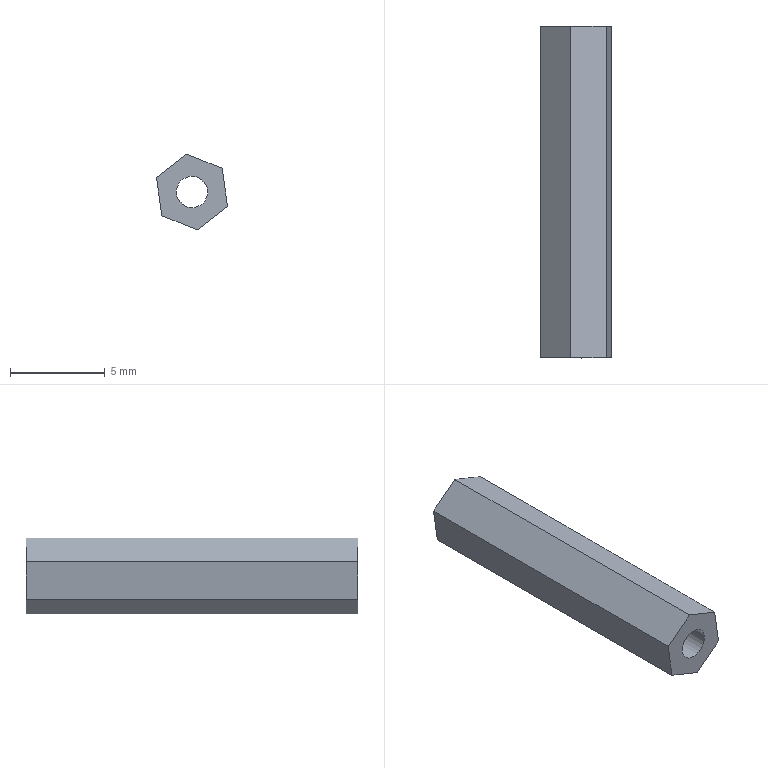Component | NX | 13 | 1 solid | 9 faces | box 3.75 x 17.5 x 4 mm | volume 148 mm3 | plane 8 | cylinder 1 | commonest cylinder face diameters 1.65 x1
STEP:
#1=CARTESIAN_POINT('',(0.,0.,0.));
#2=DIRECTION('',(0.,0.,1.));
#3=DIRECTION('',(1.,0.,0.));
#4=AXIS2_PLACEMENT_3D('',#1,#2,#3);
#5=CARTESIAN_POINT('',(-512.048,186.249,-204.937));
#6=VERTEX_POINT('',#5);
#7=CARTESIAN_POINT('',(-512.048,168.749,-204.937));
#8=VERTEX_POINT('',#7);
#9=CARTESIAN_POINT('',(-512.048,168.749,-204.937));
#10=DIRECTION('',(0.,-1.,0.));
#11=VECTOR('',#10,1.);
#12=LINE('',#9,#11);
#13=CARTESIAN_POINT('',(-510.174,168.749,-205.694));
#14=DIRECTION('',(-0.3746,0.,-0.9272));
#15=DIRECTION('',(-0.9272,0.,0.3746));
#16=AXIS2_PLACEMENT_3D('',#13,#14,#15);
#17=PLANE('',#16);
#18=CARTESIAN_POINT('',(2.021,0.));
#19=DIRECTION('',(0.,-1.));
#20=VECTOR('',#19,1.);
#21=LINE('',#18,#20);
#22=(GEOMETRIC_REPRESENTATION_CONTEXT(2)PARAMETRIC_REPRESENTATION_CONTEXT()REPRESENTATION_CONTEXT('',''));
#23=DEFINITIONAL_REPRESENTATION('',(#21),#22);
#24=PCURVE('',#17,#23);
#25=CARTESIAN_POINT('',(-512.048,168.749,-204.937));
#26=DIRECTION('',(0.6157,0.,-0.788));
#27=DIRECTION('',(0.,-1.,0.));
#28=AXIS2_PLACEMENT_3D('',#25,#26,#27);
#29=PLANE('',#28);
#30=CARTESIAN_POINT('',(0.,0.));
#31=DIRECTION('',(1.,0.));
#32=VECTOR('',#31,1.);
#33=LINE('',#30,#32);
#34=(GEOMETRIC_REPRESENTATION_CONTEXT(2)PARAMETRIC_REPRESENTATION_CONTEXT()REPRESENTATION_CONTEXT('',''));
#35=DEFINITIONAL_REPRESENTATION('',(#33),#34);
#36=PCURVE('',#29,#35);
#37=SURFACE_CURVE('',#12,(#24,#36),.PCURVE_S1.);
#38=EDGE_CURVE('',#6,#8,#37,.T.);
#39=ORIENTED_EDGE('',*,*,#38,.T.);
#40=CARTESIAN_POINT('',(-510.174,168.749,-205.694));
#41=VERTEX_POINT('',#40);
#42=CARTESIAN_POINT('',(-510.174,168.749,-205.694));
#43=DIRECTION('',(-0.9272,0.,0.3746));
#44=VECTOR('',#43,1.);
#45=LINE('',#42,#44);
#46=CARTESIAN_POINT('',(0.,0.));
#47=DIRECTION('',(1.,0.));
#48=VECTOR('',#47,1.);
#49=LINE('',#46,#48);
#50=(GEOMETRIC_REPRESENTATION_CONTEXT(2)PARAMETRIC_REPRESENTATION_CONTEXT()REPRESENTATION_CONTEXT('',''));
#51=DEFINITIONAL_REPRESENTATION('',(#49),#50);
#52=PCURVE('',#17,#51);
#53=CARTESIAN_POINT('',(-511.767,168.749,-206.939));
#54=DIRECTION('',(0.,-1.,0.));
#55=DIRECTION('',(-0.788,0.,-0.6157));
#56=AXIS2_PLACEMENT_3D('',#53,#54,#55);
#57=PLANE('',#56);
#58=CARTESIAN_POINT('',(-2.021,0.));
#59=DIRECTION('',(0.5,-0.866));
#60=VECTOR('',#59,1.);
#61=LINE('',#58,#60);
#62=(GEOMETRIC_REPRESENTATION_CONTEXT(2)PARAMETRIC_REPRESENTATION_CONTEXT()REPRESENTATION_CONTEXT('',''));
#63=DEFINITIONAL_REPRESENTATION('',(#61),#62);
#64=PCURVE('',#57,#63);
#65=SURFACE_CURVE('',#45,(#52,#64),.PCURVE_S1.);
#66=EDGE_CURVE('',#41,#8,#65,.T.);
#67=ORIENTED_EDGE('',*,*,#66,.F.);
#68=CARTESIAN_POINT('',(-510.174,186.249,-205.694));
#69=VERTEX_POINT('',#68);
#70=CARTESIAN_POINT('',(-510.174,168.749,-205.694));
#71=DIRECTION('',(0.,1.,0.));
#72=VECTOR('',#71,1.);
#73=LINE('',#70,#72);
#74=CARTESIAN_POINT('',(0.,0.));
#75=DIRECTION('',(0.,1.));
#76=VECTOR('',#75,1.);
#77=LINE('',#74,#76);
#78=(GEOMETRIC_REPRESENTATION_CONTEXT(2)PARAMETRIC_REPRESENTATION_CONTEXT()REPRESENTATION_CONTEXT('',''));
#79=DEFINITIONAL_REPRESENTATION('',(#77),#78);
#80=PCURVE('',#17,#79);
#81=CARTESIAN_POINT('',(-509.893,168.749,-207.695));
#82=DIRECTION('',(-0.9903,0.,-0.1392));
#83=DIRECTION('',(-0.1392,0.,0.9903));
#84=AXIS2_PLACEMENT_3D('',#81,#82,#83);
#85=PLANE('',#84);
#86=CARTESIAN_POINT('',(2.021,0.));
#87=DIRECTION('',(0.,1.));
#88=VECTOR('',#87,1.);
#89=LINE('',#86,#88);
#90=(GEOMETRIC_REPRESENTATION_CONTEXT(2)PARAMETRIC_REPRESENTATION_CONTEXT()REPRESENTATION_CONTEXT('',''));
#91=DEFINITIONAL_REPRESENTATION('',(#89),#90);
#92=PCURVE('',#85,#91);
#93=SURFACE_CURVE('',#73,(#80,#92),.PCURVE_S1.);
#94=EDGE_CURVE('',#41,#69,#93,.T.);
#95=ORIENTED_EDGE('',*,*,#94,.T.);
#96=CARTESIAN_POINT('',(-510.174,186.249,-205.694));
#97=DIRECTION('',(-0.9272,0.,0.3746));
#98=VECTOR('',#97,1.);
#99=LINE('',#96,#98);
#100=CARTESIAN_POINT('',(0.,17.5));
#101=DIRECTION('',(1.,0.));
#102=VECTOR('',#101,1.);
#103=LINE('',#100,#102);
#104=(GEOMETRIC_REPRESENTATION_CONTEXT(2)PARAMETRIC_REPRESENTATION_CONTEXT()REPRESENTATION_CONTEXT('',''));
#105=DEFINITIONAL_REPRESENTATION('',(#103),#104);
#106=PCURVE('',#17,#105);
#107=CARTESIAN_POINT('',(-511.767,186.249,-206.939));
#108=DIRECTION('',(0.,-1.,0.));
#109=DIRECTION('',(-0.788,0.,-0.6157));
#110=AXIS2_PLACEMENT_3D('',#107,#108,#109);
#111=PLANE('',#110);
#112=CARTESIAN_POINT('',(-2.021,0.));
#113=DIRECTION('',(0.5,-0.866));
#114=VECTOR('',#113,1.);
#115=LINE('',#112,#114);
#116=(GEOMETRIC_REPRESENTATION_CONTEXT(2)PARAMETRIC_REPRESENTATION_CONTEXT()REPRESENTATION_CONTEXT('',''));
#117=DEFINITIONAL_REPRESENTATION('',(#115),#116);
#118=PCURVE('',#111,#117);
#119=SURFACE_CURVE('',#99,(#106,#118),.PCURVE_S1.);
#120=EDGE_CURVE('',#69,#6,#119,.T.);
#121=ORIENTED_EDGE('',*,*,#120,.T.);
#122=EDGE_LOOP('',(#39,#67,#95,#121));
#123=FACE_BOUND('',#122,.T.);
#124=ADVANCED_FACE('',(#123),#17,.F.);
#125=CARTESIAN_POINT('',(-513.64,186.249,-206.182));
#126=VERTEX_POINT('',#125);
#127=CARTESIAN_POINT('',(-513.64,168.749,-206.182));
#128=VERTEX_POINT('',#127);
#129=CARTESIAN_POINT('',(-513.64,168.749,-206.182));
#130=DIRECTION('',(0.,-1.,0.));
#131=VECTOR('',#130,1.);
#132=LINE('',#129,#131);
#133=CARTESIAN_POINT('',(0.,2.021));
#134=DIRECTION('',(1.,0.));
#135=VECTOR('',#134,1.);
#136=LINE('',#133,#135);
#137=(GEOMETRIC_REPRESENTATION_CONTEXT(2)PARAMETRIC_REPRESENTATION_CONTEXT()REPRESENTATION_CONTEXT('',''));
#138=DEFINITIONAL_REPRESENTATION('',(#136),#137);
#139=PCURVE('',#29,#138);
#140=CARTESIAN_POINT('',(-513.64,168.749,-206.182));
#141=DIRECTION('',(0.9903,0.,0.1392));
#142=DIRECTION('',(0.1392,0.,-0.9903));
#143=AXIS2_PLACEMENT_3D('',#140,#141,#142);
#144=PLANE('',#143);
#145=CARTESIAN_POINT('',(0.,0.));
#146=DIRECTION('',(0.,-1.));
#147=VECTOR('',#146,1.);
#148=LINE('',#145,#147);
#149=(GEOMETRIC_REPRESENTATION_CONTEXT(2)PARAMETRIC_REPRESENTATION_CONTEXT()REPRESENTATION_CONTEXT('',''));
#150=DEFINITIONAL_REPRESENTATION('',(#148),#149);
#151=PCURVE('',#144,#150);
#152=SURFACE_CURVE('',#132,(#139,#151),.PCURVE_S1.);
#153=EDGE_CURVE('',#126,#128,#152,.T.);
#154=ORIENTED_EDGE('',*,*,#153,.T.);
#155=CARTESIAN_POINT('',(-512.844,168.749,-205.559));
#156=DIRECTION('',(-0.788,0.,-0.6157));
#157=VECTOR('',#156,1.);
#158=LINE('',#155,#157);
#159=CARTESIAN_POINT('',(0.,1.01));
#160=DIRECTION('',(0.,1.));
#161=VECTOR('',#160,1.);
#162=LINE('',#159,#161);
#163=(GEOMETRIC_REPRESENTATION_CONTEXT(2)PARAMETRIC_REPRESENTATION_CONTEXT()REPRESENTATION_CONTEXT('',''));
#164=DEFINITIONAL_REPRESENTATION('',(#162),#163);
#165=PCURVE('',#29,#164);
#166=CARTESIAN_POINT('',(0.,-1.75));
#167=DIRECTION('',(1.,0.));
#168=VECTOR('',#167,1.);
#169=LINE('',#166,#168);
#170=(GEOMETRIC_REPRESENTATION_CONTEXT(2)PARAMETRIC_REPRESENTATION_CONTEXT()REPRESENTATION_CONTEXT('',''));
#171=DEFINITIONAL_REPRESENTATION('',(#169),#170);
#172=PCURVE('',#57,#171);
#173=SURFACE_CURVE('',#158,(#165,#172),.PCURVE_S1.);
#174=EDGE_CURVE('',#8,#128,#173,.T.);
#175=ORIENTED_EDGE('',*,*,#174,.F.);
#176=ORIENTED_EDGE('',*,*,#38,.F.);
#177=CARTESIAN_POINT('',(-512.844,186.249,-205.559));
#178=DIRECTION('',(-0.788,0.,-0.6157));
#179=VECTOR('',#178,1.);
#180=LINE('',#177,#179);
#181=CARTESIAN_POINT('',(-17.5,1.01));
#182=DIRECTION('',(0.,1.));
#183=VECTOR('',#182,1.);
#184=LINE('',#181,#183);
#185=(GEOMETRIC_REPRESENTATION_CONTEXT(2)PARAMETRIC_REPRESENTATION_CONTEXT()REPRESENTATION_CONTEXT('',''));
#186=DEFINITIONAL_REPRESENTATION('',(#184),#185);
#187=PCURVE('',#29,#186);
#188=CARTESIAN_POINT('',(0.,-1.75));
#189=DIRECTION('',(1.,0.));
#190=VECTOR('',#189,1.);
#191=LINE('',#188,#190);
#192=(GEOMETRIC_REPRESENTATION_CONTEXT(2)PARAMETRIC_REPRESENTATION_CONTEXT()REPRESENTATION_CONTEXT('',''));
#193=DEFINITIONAL_REPRESENTATION('',(#191),#192);
#194=PCURVE('',#111,#193);
#195=SURFACE_CURVE('',#180,(#187,#194),.PCURVE_S1.);
#196=EDGE_CURVE('',#6,#126,#195,.T.);
#197=ORIENTED_EDGE('',*,*,#196,.T.);
#198=EDGE_LOOP('',(#154,#175,#176,#197));
#199=FACE_BOUND('',#198,.T.);
#200=ADVANCED_FACE('',(#199),#29,.F.);
#201=CARTESIAN_POINT('',(-513.359,186.249,-208.183));
#202=VERTEX_POINT('',#201);
#203=CARTESIAN_POINT('',(-513.359,168.749,-208.183));
#204=VERTEX_POINT('',#203);
#205=CARTESIAN_POINT('',(-513.359,168.749,-208.183));
#206=DIRECTION('',(0.,-1.,0.));
#207=VECTOR('',#206,1.);
#208=LINE('',#205,#207);
#209=CARTESIAN_POINT('',(2.021,0.));
#210=DIRECTION('',(0.,-1.));
#211=VECTOR('',#210,1.);
#212=LINE('',#209,#211);
#213=(GEOMETRIC_REPRESENTATION_CONTEXT(2)PARAMETRIC_REPRESENTATION_CONTEXT()REPRESENTATION_CONTEXT('',''));
#214=DEFINITIONAL_REPRESENTATION('',(#212),#213);
#215=PCURVE('',#144,#214);
#216=CARTESIAN_POINT('',(-513.359,168.749,-208.183));
#217=DIRECTION('',(0.3746,0.,0.9272));
#218=DIRECTION('',(0.9272,0.,-0.3746));
#219=AXIS2_PLACEMENT_3D('',#216,#217,#218);
#220=PLANE('',#219);
#221=CARTESIAN_POINT('',(0.,0.));
#222=DIRECTION('',(0.,-1.));
#223=VECTOR('',#222,1.);
#224=LINE('',#221,#223);
#225=(GEOMETRIC_REPRESENTATION_CONTEXT(2)PARAMETRIC_REPRESENTATION_CONTEXT()REPRESENTATION_CONTEXT('',''));
#226=DEFINITIONAL_REPRESENTATION('',(#224),#225);
#227=PCURVE('',#220,#226);
#228=SURFACE_CURVE('',#208,(#215,#227),.PCURVE_S1.);
#229=EDGE_CURVE('',#202,#204,#228,.T.);
#230=ORIENTED_EDGE('',*,*,#229,.T.);
#231=CARTESIAN_POINT('',(-513.64,168.749,-206.182));
#232=DIRECTION('',(0.1392,0.,-0.9903));
#233=VECTOR('',#232,1.);
#234=LINE('',#231,#233);
#235=CARTESIAN_POINT('',(0.,0.));
#236=DIRECTION('',(1.,0.));
#237=VECTOR('',#236,1.);
#238=LINE('',#235,#237);
#239=(GEOMETRIC_REPRESENTATION_CONTEXT(2)PARAMETRIC_REPRESENTATION_CONTEXT()REPRESENTATION_CONTEXT('',''));
#240=DEFINITIONAL_REPRESENTATION('',(#238),#239);
#241=PCURVE('',#144,#240);
#242=CARTESIAN_POINT('',(1.01,-1.75));
#243=DIRECTION('',(0.5,0.866));
#244=VECTOR('',#243,1.);
#245=LINE('',#242,#244);
#246=(GEOMETRIC_REPRESENTATION_CONTEXT(2)PARAMETRIC_REPRESENTATION_CONTEXT()REPRESENTATION_CONTEXT('',''));
#247=DEFINITIONAL_REPRESENTATION('',(#245),#246);
#248=PCURVE('',#57,#247);
#249=SURFACE_CURVE('',#234,(#241,#248),.PCURVE_S1.);
#250=EDGE_CURVE('',#128,#204,#249,.T.);
#251=ORIENTED_EDGE('',*,*,#250,.F.);
#252=ORIENTED_EDGE('',*,*,#153,.F.);
#253=CARTESIAN_POINT('',(-513.64,186.249,-206.182));
#254=DIRECTION('',(0.1392,0.,-0.9903));
#255=VECTOR('',#254,1.);
#256=LINE('',#253,#255);
#257=CARTESIAN_POINT('',(0.,17.5));
#258=DIRECTION('',(1.,0.));
#259=VECTOR('',#258,1.);
#260=LINE('',#257,#259);
#261=(GEOMETRIC_REPRESENTATION_CONTEXT(2)PARAMETRIC_REPRESENTATION_CONTEXT()REPRESENTATION_CONTEXT('',''));
#262=DEFINITIONAL_REPRESENTATION('',(#260),#261);
#263=PCURVE('',#144,#262);
#264=CARTESIAN_POINT('',(1.01,-1.75));
#265=DIRECTION('',(0.5,0.866));
#266=VECTOR('',#265,1.);
#267=LINE('',#264,#266);
#268=(GEOMETRIC_REPRESENTATION_CONTEXT(2)PARAMETRIC_REPRESENTATION_CONTEXT()REPRESENTATION_CONTEXT('',''));
#269=DEFINITIONAL_REPRESENTATION('',(#267),#268);
#270=PCURVE('',#111,#269);
#271=SURFACE_CURVE('',#256,(#263,#270),.PCURVE_S1.);
#272=EDGE_CURVE('',#126,#202,#271,.T.);
#273=ORIENTED_EDGE('',*,*,#272,.T.);
#274=EDGE_LOOP('',(#230,#251,#252,#273));
#275=FACE_BOUND('',#274,.T.);
#276=ADVANCED_FACE('',(#275),#144,.F.);
#277=CARTESIAN_POINT('',(-511.485,186.249,-208.94));
#278=VERTEX_POINT('',#277);
#279=CARTESIAN_POINT('',(-511.485,168.749,-208.94));
#280=VERTEX_POINT('',#279);
#281=CARTESIAN_POINT('',(-511.485,168.749,-208.94));
#282=DIRECTION('',(0.,-1.,0.));
#283=VECTOR('',#282,1.);
#284=LINE('',#281,#283);
#285=CARTESIAN_POINT('',(2.021,0.));
#286=DIRECTION('',(0.,-1.));
#287=VECTOR('',#286,1.);
#288=LINE('',#285,#287);
#289=(GEOMETRIC_REPRESENTATION_CONTEXT(2)PARAMETRIC_REPRESENTATION_CONTEXT()REPRESENTATION_CONTEXT('',''));
#290=DEFINITIONAL_REPRESENTATION('',(#288),#289);
#291=PCURVE('',#220,#290);
#292=CARTESIAN_POINT('',(-511.485,168.749,-208.94));
#293=DIRECTION('',(-0.6157,0.,0.788));
#294=DIRECTION('',(0.788,0.,0.6157));
#295=AXIS2_PLACEMENT_3D('',#292,#293,#294);
#296=PLANE('',#295);
#297=CARTESIAN_POINT('',(0.,0.));
#298=DIRECTION('',(0.,-1.));
#299=VECTOR('',#298,1.);
#300=LINE('',#297,#299);
#301=(GEOMETRIC_REPRESENTATION_CONTEXT(2)PARAMETRIC_REPRESENTATION_CONTEXT()REPRESENTATION_CONTEXT('',''));
#302=DEFINITIONAL_REPRESENTATION('',(#300),#301);
#303=PCURVE('',#296,#302);
#304=SURFACE_CURVE('',#284,(#291,#303),.PCURVE_S1.);
#305=EDGE_CURVE('',#278,#280,#304,.T.);
#306=ORIENTED_EDGE('',*,*,#305,.T.);
#307=CARTESIAN_POINT('',(-513.359,168.749,-208.183));
#308=DIRECTION('',(0.9272,0.,-0.3746));
#309=VECTOR('',#308,1.);
#310=LINE('',#307,#309);
#311=CARTESIAN_POINT('',(0.,0.));
#312=DIRECTION('',(1.,0.));
#313=VECTOR('',#312,1.);
#314=LINE('',#311,#313);
#315=(GEOMETRIC_REPRESENTATION_CONTEXT(2)PARAMETRIC_REPRESENTATION_CONTEXT()REPRESENTATION_CONTEXT('',''));
#316=DEFINITIONAL_REPRESENTATION('',(#314),#315);
#317=PCURVE('',#220,#316);
#318=CARTESIAN_POINT('',(2.021,0.));
#319=DIRECTION('',(-0.5,0.866));
#320=VECTOR('',#319,1.);
#321=LINE('',#318,#320);
#322=(GEOMETRIC_REPRESENTATION_CONTEXT(2)PARAMETRIC_REPRESENTATION_CONTEXT()REPRESENTATION_CONTEXT('',''));
#323=DEFINITIONAL_REPRESENTATION('',(#321),#322);
#324=PCURVE('',#57,#323);
#325=SURFACE_CURVE('',#310,(#317,#324),.PCURVE_S1.);
#326=EDGE_CURVE('',#204,#280,#325,.T.);
#327=ORIENTED_EDGE('',*,*,#326,.F.);
#328=ORIENTED_EDGE('',*,*,#229,.F.);
#329=CARTESIAN_POINT('',(-513.359,186.249,-208.183));
#330=DIRECTION('',(0.9272,0.,-0.3746));
#331=VECTOR('',#330,1.);
#332=LINE('',#329,#331);
#333=CARTESIAN_POINT('',(0.,17.5));
#334=DIRECTION('',(1.,0.));
#335=VECTOR('',#334,1.);
#336=LINE('',#333,#335);
#337=(GEOMETRIC_REPRESENTATION_CONTEXT(2)PARAMETRIC_REPRESENTATION_CONTEXT()REPRESENTATION_CONTEXT('',''));
#338=DEFINITIONAL_REPRESENTATION('',(#336),#337);
#339=PCURVE('',#220,#338);
#340=CARTESIAN_POINT('',(2.021,0.));
#341=DIRECTION('',(-0.5,0.866));
#342=VECTOR('',#341,1.);
#343=LINE('',#340,#342);
#344=(GEOMETRIC_REPRESENTATION_CONTEXT(2)PARAMETRIC_REPRESENTATION_CONTEXT()REPRESENTATION_CONTEXT('',''));
#345=DEFINITIONAL_REPRESENTATION('',(#343),#344);
#346=PCURVE('',#111,#345);
#347=SURFACE_CURVE('',#332,(#339,#346),.PCURVE_S1.);
#348=EDGE_CURVE('',#202,#278,#347,.T.);
#349=ORIENTED_EDGE('',*,*,#348,.T.);
#350=EDGE_LOOP('',(#306,#327,#328,#349));
#351=FACE_BOUND('',#350,.T.);
#352=ADVANCED_FACE('',(#351),#220,.F.);
#353=CARTESIAN_POINT('',(-509.893,186.249,-207.695));
#354=VERTEX_POINT('',#353);
#355=CARTESIAN_POINT('',(-509.893,168.749,-207.695));
#356=VERTEX_POINT('',#355);
#357=CARTESIAN_POINT('',(-509.893,168.749,-207.695));
#358=DIRECTION('',(0.,-1.,0.));
#359=VECTOR('',#358,1.);
#360=LINE('',#357,#359);
#361=CARTESIAN_POINT('',(2.021,0.));
#362=DIRECTION('',(0.,-1.));
#363=VECTOR('',#362,1.);
#364=LINE('',#361,#363);
#365=(GEOMETRIC_REPRESENTATION_CONTEXT(2)PARAMETRIC_REPRESENTATION_CONTEXT()REPRESENTATION_CONTEXT('',''));
#366=DEFINITIONAL_REPRESENTATION('',(#364),#365);
#367=PCURVE('',#296,#366);
#368=CARTESIAN_POINT('',(0.,0.));
#369=DIRECTION('',(0.,-1.));
#370=VECTOR('',#369,1.);
#371=LINE('',#368,#370);
#372=(GEOMETRIC_REPRESENTATION_CONTEXT(2)PARAMETRIC_REPRESENTATION_CONTEXT()REPRESENTATION_CONTEXT('',''));
#373=DEFINITIONAL_REPRESENTATION('',(#371),#372);
#374=PCURVE('',#85,#373);
#375=SURFACE_CURVE('',#360,(#367,#374),.PCURVE_S1.);
#376=EDGE_CURVE('',#354,#356,#375,.T.);
#377=ORIENTED_EDGE('',*,*,#376,.T.);
#378=CARTESIAN_POINT('',(-510.689,168.749,-208.318));
#379=DIRECTION('',(0.788,0.,0.6157));
#380=VECTOR('',#379,1.);
#381=LINE('',#378,#380);
#382=CARTESIAN_POINT('',(1.01,0.));
#383=DIRECTION('',(1.,0.));
#384=VECTOR('',#383,1.);
#385=LINE('',#382,#384);
#386=(GEOMETRIC_REPRESENTATION_CONTEXT(2)PARAMETRIC_REPRESENTATION_CONTEXT()REPRESENTATION_CONTEXT('',''));
#387=DEFINITIONAL_REPRESENTATION('',(#385),#386);
#388=PCURVE('',#296,#387);
#389=CARTESIAN_POINT('',(-0.,1.75));
#390=DIRECTION('',(-1.,0.));
#391=VECTOR('',#390,1.);
#392=LINE('',#389,#391);
#393=(GEOMETRIC_REPRESENTATION_CONTEXT(2)PARAMETRIC_REPRESENTATION_CONTEXT()REPRESENTATION_CONTEXT('',''));
#394=DEFINITIONAL_REPRESENTATION('',(#392),#393);
#395=PCURVE('',#57,#394);
#396=SURFACE_CURVE('',#381,(#388,#395),.PCURVE_S1.);
#397=EDGE_CURVE('',#280,#356,#396,.T.);
#398=ORIENTED_EDGE('',*,*,#397,.F.);
#399=ORIENTED_EDGE('',*,*,#305,.F.);
#400=CARTESIAN_POINT('',(-510.689,186.249,-208.318));
#401=DIRECTION('',(0.788,0.,0.6157));
#402=VECTOR('',#401,1.);
#403=LINE('',#400,#402);
#404=CARTESIAN_POINT('',(1.01,17.5));
#405=DIRECTION('',(1.,0.));
#406=VECTOR('',#405,1.);
#407=LINE('',#404,#406);
#408=(GEOMETRIC_REPRESENTATION_CONTEXT(2)PARAMETRIC_REPRESENTATION_CONTEXT()REPRESENTATION_CONTEXT('',''));
#409=DEFINITIONAL_REPRESENTATION('',(#407),#408);
#410=PCURVE('',#296,#409);
#411=CARTESIAN_POINT('',(-0.,1.75));
#412=DIRECTION('',(-1.,0.));
#413=VECTOR('',#412,1.);
#414=LINE('',#411,#413);
#415=(GEOMETRIC_REPRESENTATION_CONTEXT(2)PARAMETRIC_REPRESENTATION_CONTEXT()REPRESENTATION_CONTEXT('',''));
#416=DEFINITIONAL_REPRESENTATION('',(#414),#415);
#417=PCURVE('',#111,#416);
#418=SURFACE_CURVE('',#403,(#410,#417),.PCURVE_S1.);
#419=EDGE_CURVE('',#278,#354,#418,.T.);
#420=ORIENTED_EDGE('',*,*,#419,.T.);
#421=EDGE_LOOP('',(#377,#398,#399,#420));
#422=FACE_BOUND('',#421,.T.);
#423=ADVANCED_FACE('',(#422),#296,.F.);
#424=ORIENTED_EDGE('',*,*,#94,.F.);
#425=CARTESIAN_POINT('',(-509.893,168.749,-207.695));
#426=DIRECTION('',(-0.1392,0.,0.9903));
#427=VECTOR('',#426,1.);
#428=LINE('',#425,#427);
#429=CARTESIAN_POINT('',(0.,0.));
#430=DIRECTION('',(1.,0.));
#431=VECTOR('',#430,1.);
#432=LINE('',#429,#431);
#433=(GEOMETRIC_REPRESENTATION_CONTEXT(2)PARAMETRIC_REPRESENTATION_CONTEXT()REPRESENTATION_CONTEXT('',''));
#434=DEFINITIONAL_REPRESENTATION('',(#432),#433);
#435=PCURVE('',#85,#434);
#436=CARTESIAN_POINT('',(-1.01,1.75));
#437=DIRECTION('',(-0.5,-0.866));
#438=VECTOR('',#437,1.);
#439=LINE('',#436,#438);
#440=(GEOMETRIC_REPRESENTATION_CONTEXT(2)PARAMETRIC_REPRESENTATION_CONTEXT()REPRESENTATION_CONTEXT('',''));
#441=DEFINITIONAL_REPRESENTATION('',(#439),#440);
#442=PCURVE('',#57,#441);
#443=SURFACE_CURVE('',#428,(#435,#442),.PCURVE_S1.);
#444=EDGE_CURVE('',#356,#41,#443,.T.);
#445=ORIENTED_EDGE('',*,*,#444,.F.);
#446=ORIENTED_EDGE('',*,*,#376,.F.);
#447=CARTESIAN_POINT('',(-509.893,186.249,-207.695));
#448=DIRECTION('',(-0.1392,0.,0.9903));
#449=VECTOR('',#448,1.);
#450=LINE('',#447,#449);
#451=CARTESIAN_POINT('',(0.,17.5));
#452=DIRECTION('',(1.,0.));
#453=VECTOR('',#452,1.);
#454=LINE('',#451,#453);
#455=(GEOMETRIC_REPRESENTATION_CONTEXT(2)PARAMETRIC_REPRESENTATION_CONTEXT()REPRESENTATION_CONTEXT('',''));
#456=DEFINITIONAL_REPRESENTATION('',(#454),#455);
#457=PCURVE('',#85,#456);
#458=CARTESIAN_POINT('',(-1.01,1.75));
#459=DIRECTION('',(-0.5,-0.866));
#460=VECTOR('',#459,1.);
#461=LINE('',#458,#460);
#462=(GEOMETRIC_REPRESENTATION_CONTEXT(2)PARAMETRIC_REPRESENTATION_CONTEXT()REPRESENTATION_CONTEXT('',''));
#463=DEFINITIONAL_REPRESENTATION('',(#461),#462);
#464=PCURVE('',#111,#463);
#465=SURFACE_CURVE('',#450,(#457,#464),.PCURVE_S1.);
#466=EDGE_CURVE('',#354,#69,#465,.T.);
#467=ORIENTED_EDGE('',*,*,#466,.T.);
#468=EDGE_LOOP('',(#424,#445,#446,#467));
#469=FACE_BOUND('',#468,.T.);
#470=ADVANCED_FACE('',(#469),#85,.F.);
#471=ORIENTED_EDGE('',*,*,#326,.T.);
#472=ORIENTED_EDGE('',*,*,#397,.T.);
#473=ORIENTED_EDGE('',*,*,#444,.T.);
#474=ORIENTED_EDGE('',*,*,#66,.T.);
#475=ORIENTED_EDGE('',*,*,#174,.T.);
#476=ORIENTED_EDGE('',*,*,#250,.T.);
#477=EDGE_LOOP('',(#471,#472,#473,#474,#475,#476));
#478=FACE_BOUND('',#477,.T.);
#479=CARTESIAN_POINT('',(-511.116,168.749,-206.431));
#480=VERTEX_POINT('',#479);
#481=CARTESIAN_POINT('',(-511.767,168.749,-206.939));
#482=DIRECTION('',(0.,1.,0.));
#483=DIRECTION('',(0.788,0.,0.6157));
#484=AXIS2_PLACEMENT_3D('',#481,#482,#483);
#485=CIRCLE('',#484,0.825);
#486=CARTESIAN_POINT('',(-0.825,-0.));
#487=CARTESIAN_POINT('',(-0.825,1.429));
#488=CARTESIAN_POINT('',(0.4125,0.7145));
#489=CARTESIAN_POINT('',(1.65,0.));
#490=CARTESIAN_POINT('',(0.4125,-0.7145));
#491=CARTESIAN_POINT('',(-0.825,-1.429));
#492=CARTESIAN_POINT('',(-0.825,-0.));
#493=(BOUNDED_CURVE()B_SPLINE_CURVE(2,(#486,#487,#488,#489,#490,#491,#492),.UNSPECIFIED.,.T.,.F.)B_SPLINE_CURVE_WITH_KNOTS((1,2,2,2,2,1),(-2.094,0.,2.094,4.189,6.283,8.378),.UNSPECIFIED.)CURVE()GEOMETRIC_REPRESENTATION_ITEM()RATIONAL_B_SPLINE_CURVE((1.,0.5,1.,0.5,1.,0.5,1.))REPRESENTATION_ITEM(''));
#494=(GEOMETRIC_REPRESENTATION_CONTEXT(2)PARAMETRIC_REPRESENTATION_CONTEXT()REPRESENTATION_CONTEXT('',''));
#495=DEFINITIONAL_REPRESENTATION('',(#493),#494);
#496=PCURVE('',#57,#495);
#497=CARTESIAN_POINT('',(-511.767,168.749,-206.939));
#498=DIRECTION('',(0.,-1.,0.));
#499=DIRECTION('',(-0.788,0.,-0.6157));
#500=AXIS2_PLACEMENT_3D('',#497,#498,#499);
#501=CYLINDRICAL_SURFACE('',#500,0.825);
#502=CARTESIAN_POINT('',(9.425,0.));
#503=DIRECTION('',(-1.,0.));
#504=VECTOR('',#503,1.);
#505=LINE('',#502,#504);
#506=(GEOMETRIC_REPRESENTATION_CONTEXT(2)PARAMETRIC_REPRESENTATION_CONTEXT()REPRESENTATION_CONTEXT('',''));
#507=DEFINITIONAL_REPRESENTATION('',(#505),#506);
#508=PCURVE('',#501,#507);
#509=SURFACE_CURVE('',#485,(#496,#508),.PCURVE_S1.);
#510=EDGE_CURVE('',#480,#480,#509,.T.);
#511=ORIENTED_EDGE('',*,*,#510,.T.);
#512=EDGE_LOOP('',(#511));
#513=FACE_BOUND('',#512,.T.);
#514=ADVANCED_FACE('',(#478,#513),#57,.T.);
#515=ORIENTED_EDGE('',*,*,#419,.F.);
#516=ORIENTED_EDGE('',*,*,#348,.F.);
#517=ORIENTED_EDGE('',*,*,#272,.F.);
#518=ORIENTED_EDGE('',*,*,#196,.F.);
#519=ORIENTED_EDGE('',*,*,#120,.F.);
#520=ORIENTED_EDGE('',*,*,#466,.F.);
#521=EDGE_LOOP('',(#515,#516,#517,#518,#519,#520));
#522=FACE_BOUND('',#521,.T.);
#523=CARTESIAN_POINT('',(-511.116,186.249,-206.431));
#524=VERTEX_POINT('',#523);
#525=CARTESIAN_POINT('',(-511.767,186.249,-206.939));
#526=DIRECTION('',(0.,-1.,0.));
#527=DIRECTION('',(0.788,0.,0.6157));
#528=AXIS2_PLACEMENT_3D('',#525,#526,#527);
#529=CIRCLE('',#528,0.825);
#530=CARTESIAN_POINT('',(0.,0.));
#531=DIRECTION('',(-1.,-0.));
#532=AXIS2_PLACEMENT_2D('',#530,#531);
#533=CIRCLE('',#532,0.825);
#534=(GEOMETRIC_REPRESENTATION_CONTEXT(2)PARAMETRIC_REPRESENTATION_CONTEXT()REPRESENTATION_CONTEXT('',''));
#535=DEFINITIONAL_REPRESENTATION('',(#533),#534);
#536=PCURVE('',#111,#535);
#537=CARTESIAN_POINT('',(3.142,-17.5));
#538=DIRECTION('',(1.,0.));
#539=VECTOR('',#538,1.);
#540=LINE('',#537,#539);
#541=(GEOMETRIC_REPRESENTATION_CONTEXT(2)PARAMETRIC_REPRESENTATION_CONTEXT()REPRESENTATION_CONTEXT('',''));
#542=DEFINITIONAL_REPRESENTATION('',(#540),#541);
#543=PCURVE('',#501,#542);
#544=SURFACE_CURVE('',#529,(#536,#543),.PCURVE_S1.);
#545=EDGE_CURVE('',#524,#524,#544,.T.);
#546=ORIENTED_EDGE('',*,*,#545,.T.);
#547=EDGE_LOOP('',(#546));
#548=FACE_BOUND('',#547,.T.);
#549=ADVANCED_FACE('',(#522,#548),#111,.F.);
#550=ORIENTED_EDGE('',*,*,#510,.T.);
#551=CARTESIAN_POINT('',(-511.116,186.249,-206.431));
#552=CARTESIAN_POINT('',(-511.116,168.749,-206.431));
#553=B_SPLINE_CURVE_WITH_KNOTS('',1,(#551,#552),.UNSPECIFIED.,.F.,.F.,(2,2),(-17.5,0.),.PIECEWISE_BEZIER_KNOTS.);
#554=CARTESIAN_POINT('',(3.142,0.));
#555=DIRECTION('',(0.,1.));
#556=VECTOR('',#555,1.);
#557=LINE('',#554,#556);
#558=(GEOMETRIC_REPRESENTATION_CONTEXT(2)PARAMETRIC_REPRESENTATION_CONTEXT()REPRESENTATION_CONTEXT('',''));
#559=DEFINITIONAL_REPRESENTATION('',(#557),#558);
#560=PCURVE('',#501,#559);
#561=CARTESIAN_POINT('',(9.425,0.));
#562=DIRECTION('',(0.,1.));
#563=VECTOR('',#562,1.);
#564=LINE('',#561,#563);
#565=(GEOMETRIC_REPRESENTATION_CONTEXT(2)PARAMETRIC_REPRESENTATION_CONTEXT()REPRESENTATION_CONTEXT('',''));
#566=DEFINITIONAL_REPRESENTATION('',(#564),#565);
#567=PCURVE('',#501,#566);
#568=SEAM_CURVE('',#553,(#560,#567),.PCURVE_S1.);
#569=EDGE_CURVE('',#524,#480,#568,.T.);
#570=ORIENTED_EDGE('',*,*,#569,.F.);
#571=ORIENTED_EDGE('',*,*,#545,.T.);
#572=ORIENTED_EDGE('',*,*,#569,.T.);
#573=EDGE_LOOP('',(#550,#570,#571,#572));
#574=FACE_BOUND('',#573,.F.);
#575=ADVANCED_FACE('',(#574),#501,.F.);
#576=CLOSED_SHELL('',(#124,#200,#276,#352,#423,#470,#514,#549,#575));
#577=MANIFOLD_SOLID_BREP('',#576);
#578=(LENGTH_UNIT()NAMED_UNIT(*)SI_UNIT(.MILLI.,.METRE.));
#579=UNCERTAINTY_MEASURE_WITH_UNIT(LENGTH_MEASURE(0.000001),#578,'','');
#580=(NAMED_UNIT(*)PLANE_ANGLE_UNIT()SI_UNIT($,.RADIAN.));
#581=(NAMED_UNIT(*)SI_UNIT($,.STERADIAN.)SOLID_ANGLE_UNIT());
#582=(GEOMETRIC_REPRESENTATION_CONTEXT(3)GLOBAL_UNCERTAINTY_ASSIGNED_CONTEXT((#579))GLOBAL_UNIT_ASSIGNED_CONTEXT((#578,#580,#581))REPRESENTATION_CONTEXT('',''));
#583=ADVANCED_BREP_SHAPE_REPRESENTATION('',(#4,#577),#582);